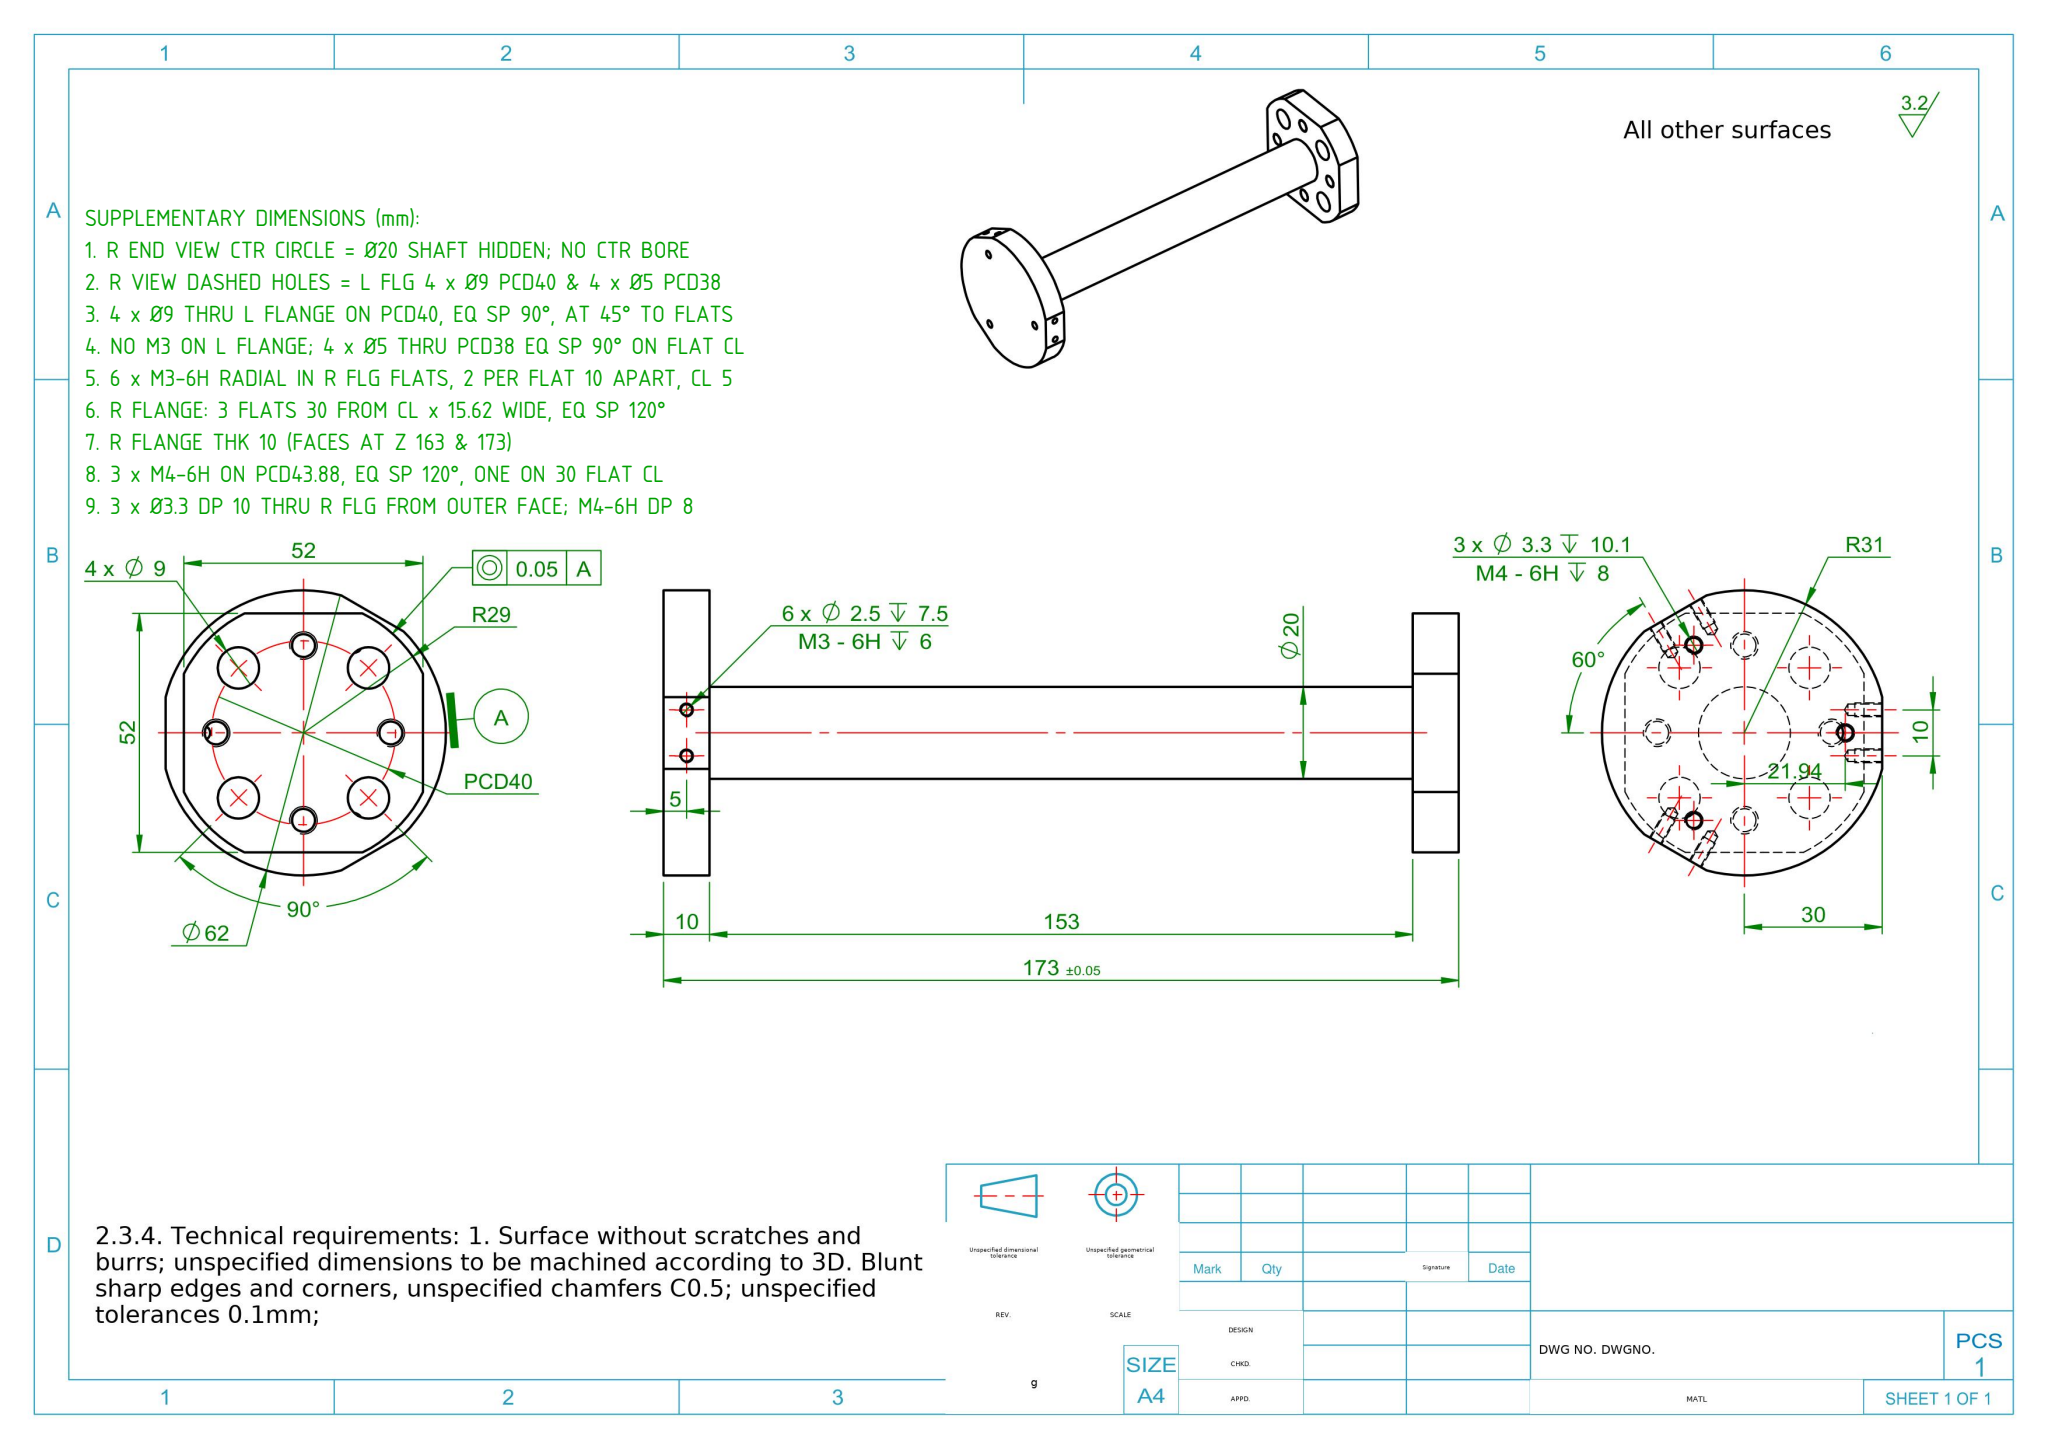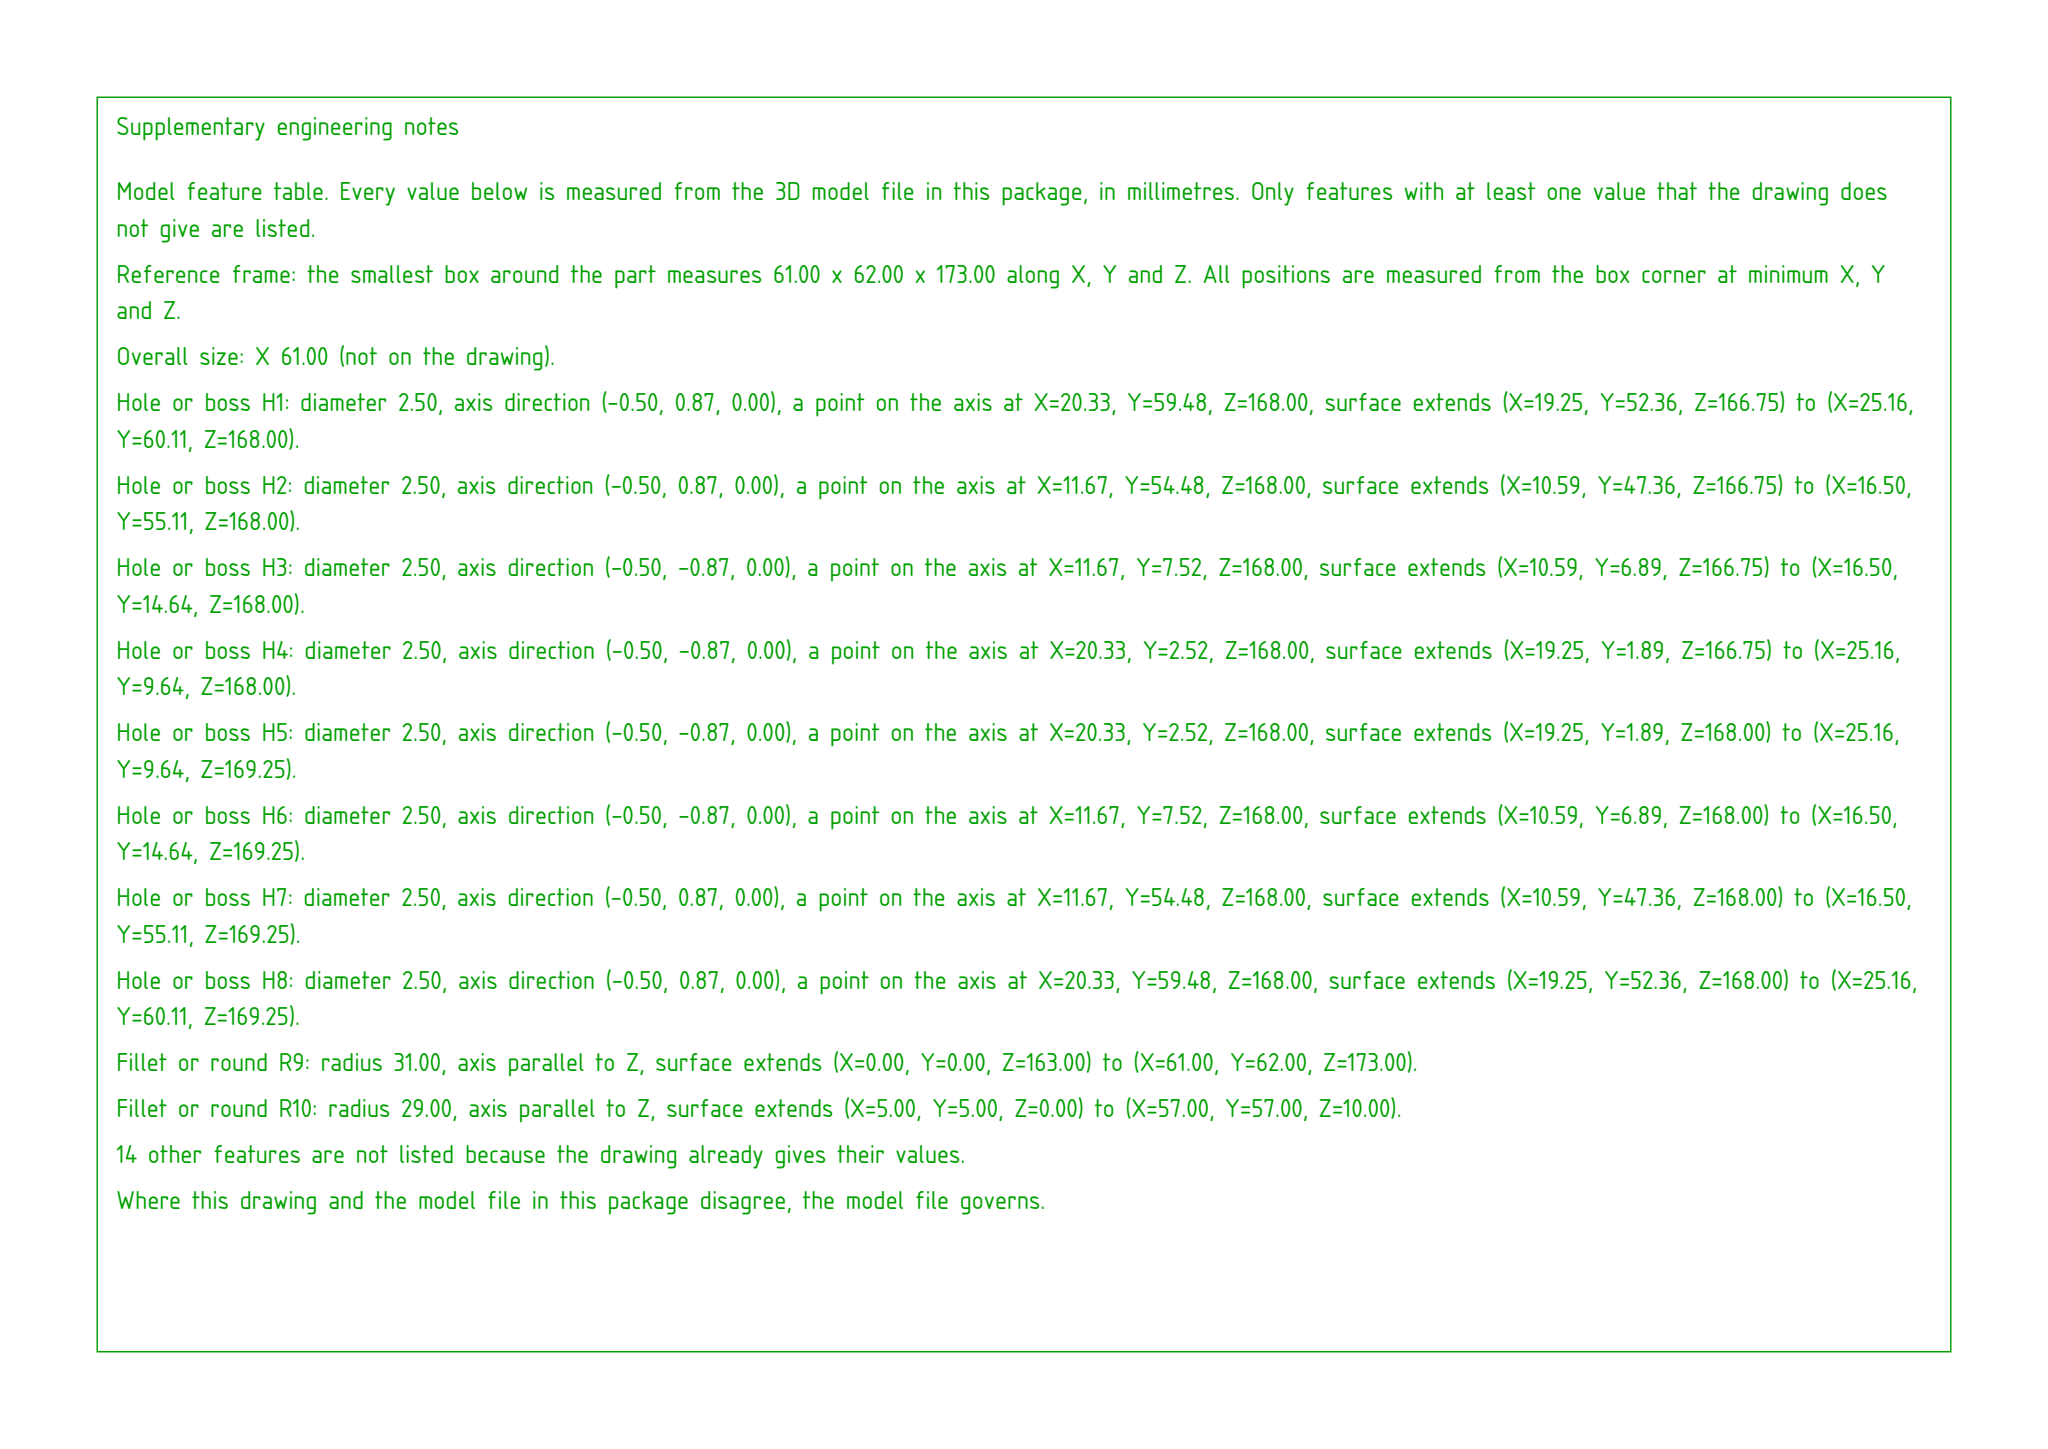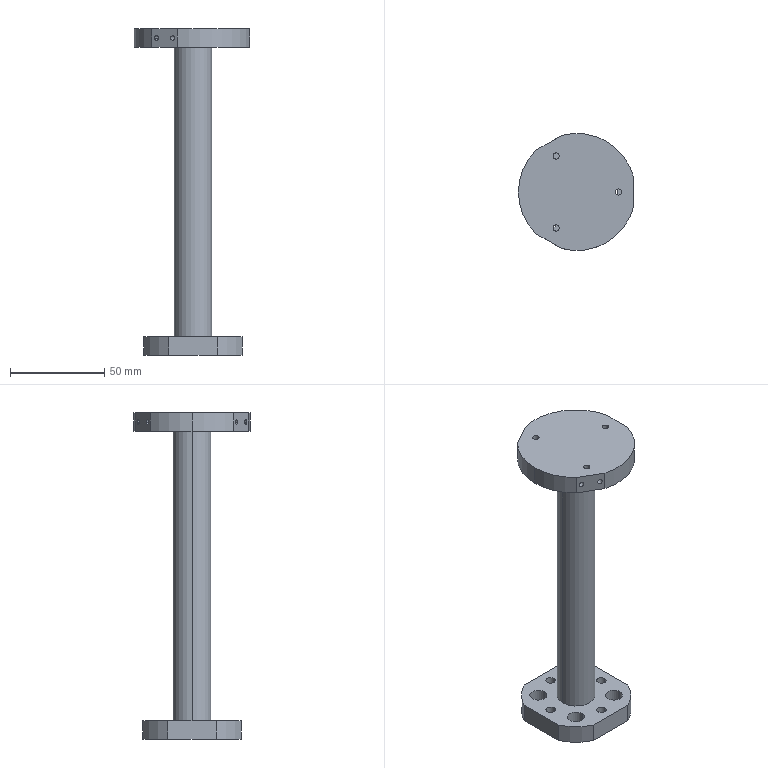Part | SolidWorks | mm | 1 solid | 67 faces | box 61 x 62 x 173 mm | volume 98472 mm3 | cylinder 44 | cone 12 | plane 11 | commonest cylinder face diameters 2.5 x12 5 x8 9 x8 3.3 x6 62 x4 58 x4 20 x2